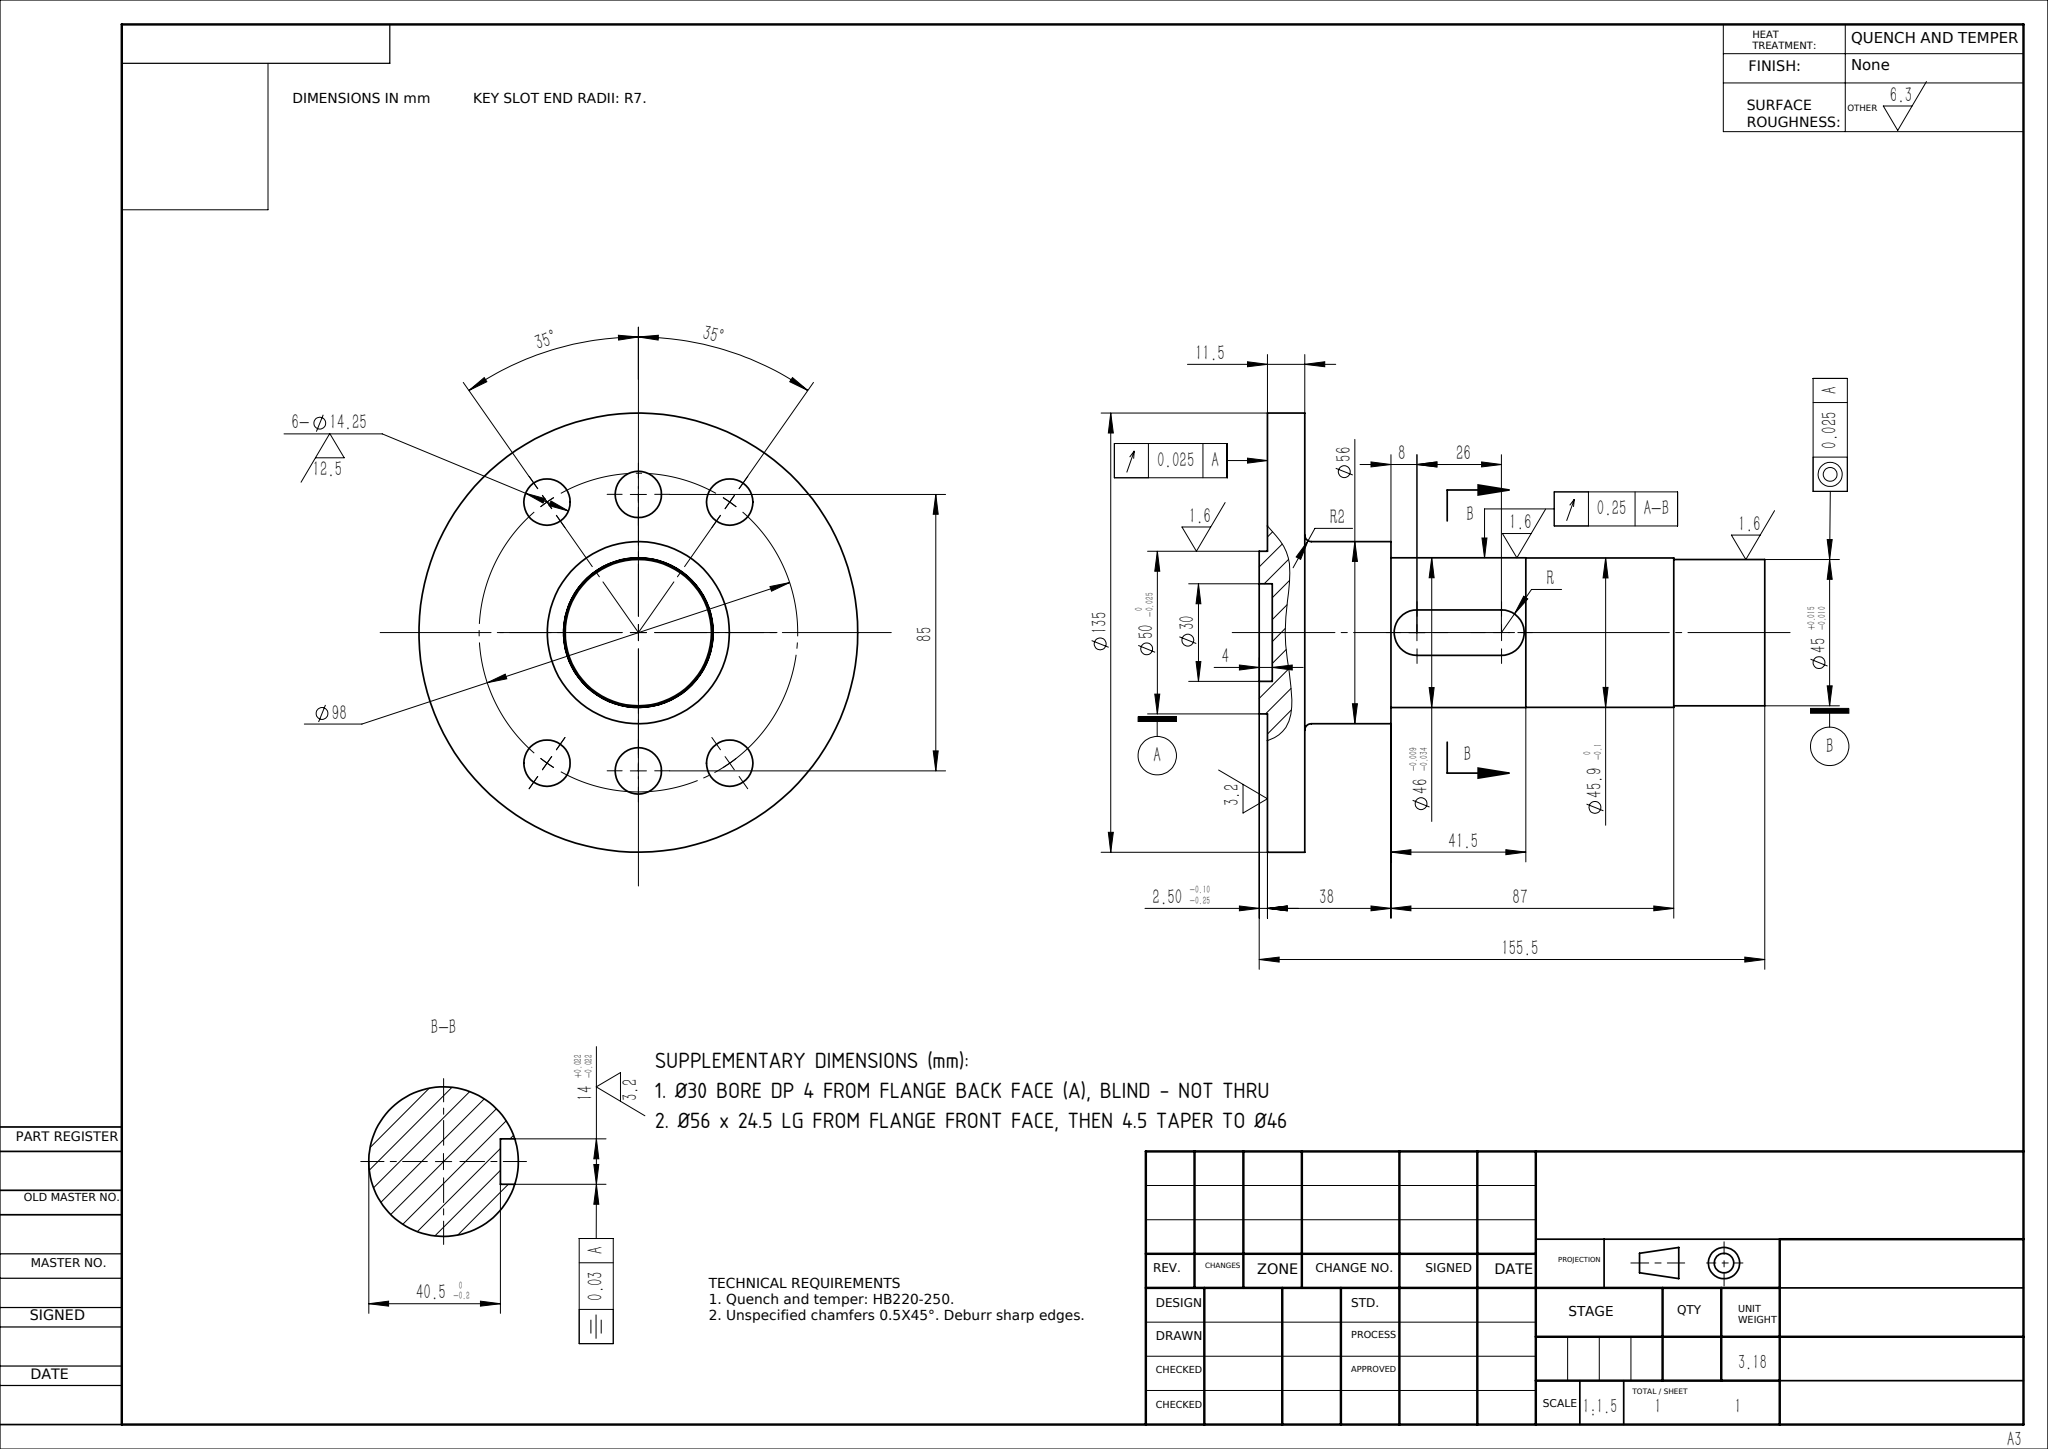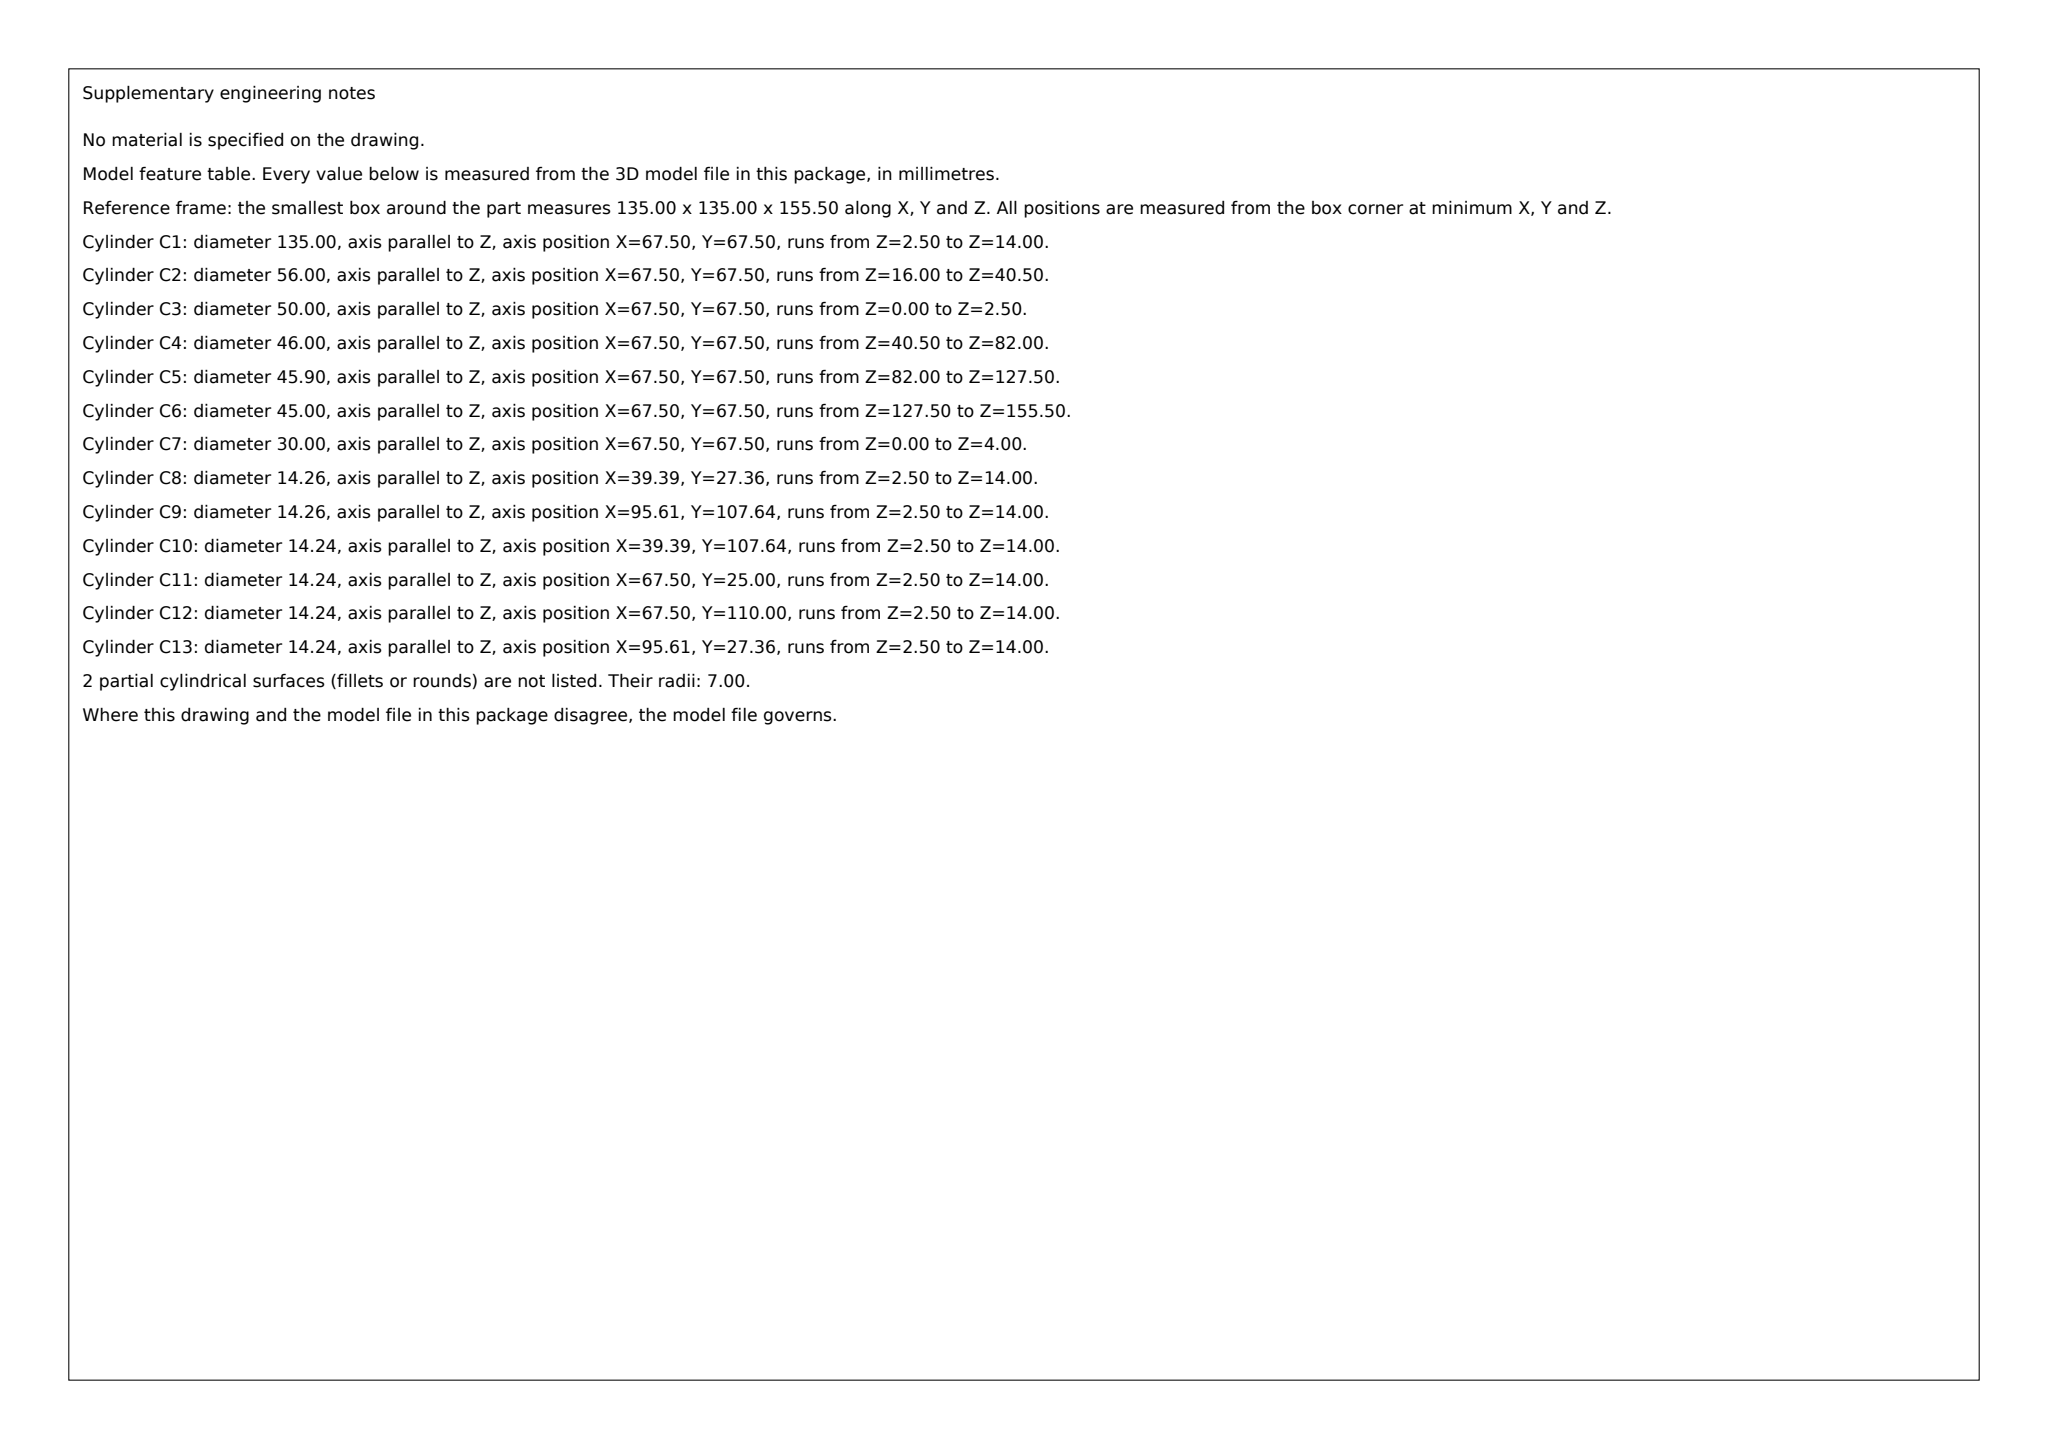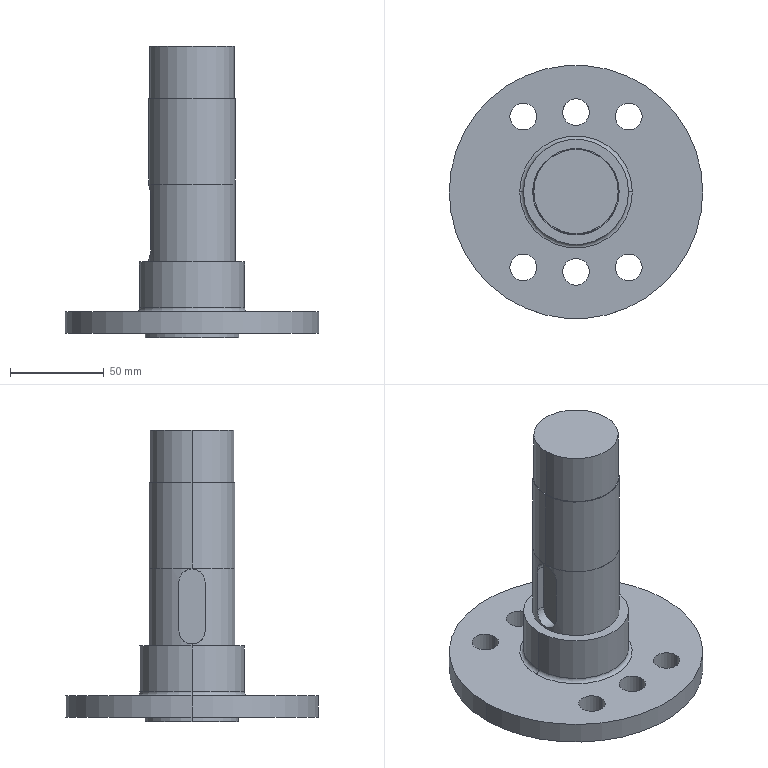Part | SolidWorks | mm | 1 solid | 42 faces | box 135 x 135 x 155.5 mm | volume 407223 mm3 | cylinder 29 | plane 11 | torus 2 | commonest cylinder face diameters 14.25 x12 14 x3 45 x2 45.9 x2 30 x2 50 x2 56 x2 135 x2
build123d program:
from build123d import *

# Parameters (mm, degrees)
SKETCH1_R           = 67.5
BOSS_EXTRUDE1_DEPTH = 14
SKETCH2_R           = 28
BOSS_EXTRUDE2_DEPTH = 26.5
SKETCH3_OUTSIDE_W   = 176.034
SKETCH3_OUTSIDE_H   = 176.034
SKETCH3_OUTSIDE_R   = 25
CUT_EXTRUDE1_DEPTH  = 2.5
SKETCH4_R           = 15
CUT_EXTRUDE2_DEPTH  = 4
SKETCH5_R           = 23
BOSS_EXTRUDE3_DEPTH = 115
SKETCH6_OUTSIDE_W   = 186.246
SKETCH6_OUTSIDE_H   = 186.246
SKETCH6_OUTSIDE_R   = 22.5
CUT_EXTRUDE3_DEPTH  = 28
SKETCH7_R           = 7.125
CUT_EXTRUDE4_DEPTH  = 171.689
CIRPATTERN1_COUNT   = 2
SKETCH8_R           = 7.125
CUT_EXTRUDE5_DEPTH  = 171.689
CUT_EXTRUDE6_DEPTH  = 5.5
SKETCH10_OUTSIDE_W  = 186.246
SKETCH10_OUTSIDE_H  = 186.246
SKETCH10_OUTSIDE_R  = 22.95
CUT_EXTRUDE7_DEPTH  = 45.5
FILLET1_R           = 2


with BuildPart() as part:
    # Sketch1 → Boss-Extrude1 (new body)
    with BuildSketch(Plane.XY):
        Circle(SKETCH1_R)
    extrude(amount=BOSS_EXTRUDE1_DEPTH)

    # Sketch2 → Boss-Extrude2 (add)
    with BuildSketch(Plane.XY.offset(14)):
        Circle(SKETCH2_R)
    extrude(amount=BOSS_EXTRUDE2_DEPTH)

    # Sketch3 outside → Cut-Extrude1 (cut)
    with BuildSketch(Plane(origin=(0, 0, 0), x_dir=(-1, 0, 0), z_dir=(0, 0, -1))):
        Rectangle(SKETCH3_OUTSIDE_W, SKETCH3_OUTSIDE_H)
        Circle(SKETCH3_OUTSIDE_R, mode=Mode.SUBTRACT)
    extrude(amount=-CUT_EXTRUDE1_DEPTH, mode=Mode.SUBTRACT)

    # Sketch4 → Cut-Extrude2 (cut)
    with BuildSketch(Plane(origin=(0, 0, 0), x_dir=(-1, 0, 0), z_dir=(0, 0, -1))):
        Circle(SKETCH4_R)
    extrude(amount=-CUT_EXTRUDE2_DEPTH, mode=Mode.SUBTRACT)

    # Sketch5 → Boss-Extrude3 (add)
    with BuildSketch(Plane.XY.offset(40.5)):
        Circle(SKETCH5_R)
    extrude(amount=BOSS_EXTRUDE3_DEPTH)

    # Sketch6 outside → Cut-Extrude3 (cut)
    with BuildSketch(Plane.XY.offset(155.5)):
        Rectangle(SKETCH6_OUTSIDE_W, SKETCH6_OUTSIDE_H)
        Circle(SKETCH6_OUTSIDE_R, mode=Mode.SUBTRACT)
    extrude(amount=-CUT_EXTRUDE3_DEPTH, mode=Mode.SUBTRACT)

    # Sketch7 → Cut-Extrude4 (cut, through all)
    with BuildSketch(Plane.XY.offset(14)):
        with Locations((-28.105, 40.138)):
            Circle(SKETCH7_R)
        with Locations((28.105, 40.138)):
            Circle(SKETCH7_R)
    cut_extrude4 = extrude(amount=-CUT_EXTRUDE4_DEPTH, mode=Mode.SUBTRACT)

    # CirPattern1: Cut-Extrude4 ×2 about axis
    cirpattern1_axis = Axis((0, 0, 0), (0, 0, 1))
    for i in range(1, CIRPATTERN1_COUNT):
        add(cut_extrude4.rotate(cirpattern1_axis, i * 360 / CIRPATTERN1_COUNT), mode=Mode.SUBTRACT)

    # Sketch8 → Cut-Extrude5 (cut, through all)
    with BuildSketch(Plane.XY.offset(14)):
        with Locations((0, 42.5)):
            Circle(SKETCH8_R)
        with Locations((0, -42.5)):
            Circle(SKETCH8_R)
    extrude(amount=-CUT_EXTRUDE5_DEPTH, mode=Mode.SUBTRACT)

    # Sketch9 → Cut-Extrude6 (cut)
    with BuildSketch(Plane.ZY.offset(23)):
        with BuildLine():
            Line((48.5, 7), (74.5, 7))
            ThreePointArc((74.5, 7), (81.5, 0), (74.5, -7))
            Line((74.5, -7), (48.5, -7))
            ThreePointArc((48.5, -7), (41.5, 0), (48.5, 7))
        make_face()
    extrude(amount=-CUT_EXTRUDE6_DEPTH, mode=Mode.SUBTRACT)

    # Sketch10 outside → Cut-Extrude7 (cut)
    with BuildSketch(Plane.XY.offset(127.5)):
        Rectangle(SKETCH10_OUTSIDE_W, SKETCH10_OUTSIDE_H)
        Circle(SKETCH10_OUTSIDE_R, mode=Mode.SUBTRACT)
    extrude(amount=-CUT_EXTRUDE7_DEPTH, mode=Mode.SUBTRACT)

    # Fillet1
    fillet1_edges = [part.edges().sort_by_distance(p)[0] for p in [
        (-28, 0, 14),
    ]]
    fillet(fillet1_edges, radius=FILLET1_R)


solid = part.part